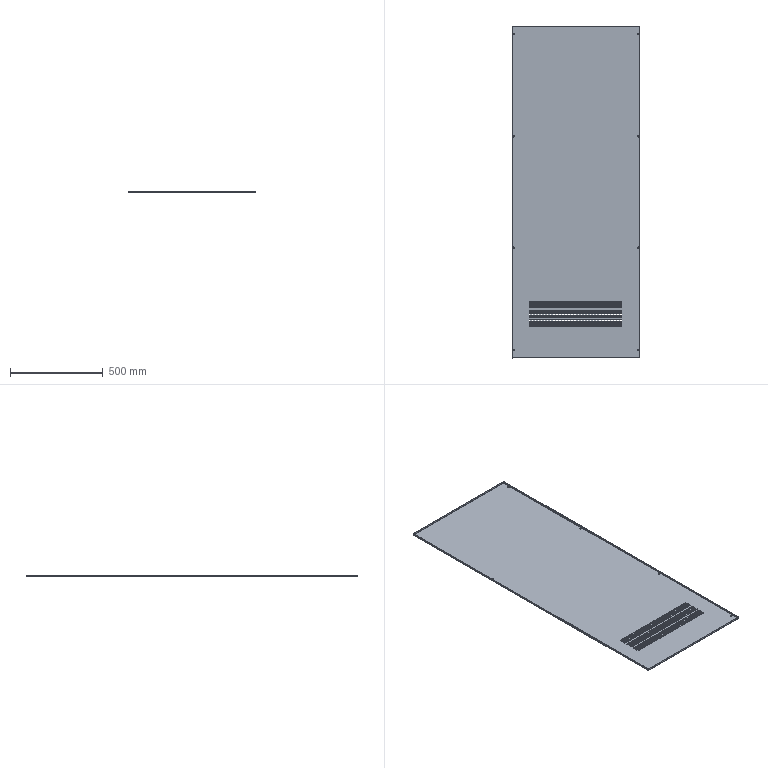Component | SolidWorks | KSHE-016.018-1 | 1 solid | 814 faces | volume 1500535 mm3 | plane 790 | cylinder 24 | commonest cylinder face diameters 7 x16 2.6 x4 0.2 x4